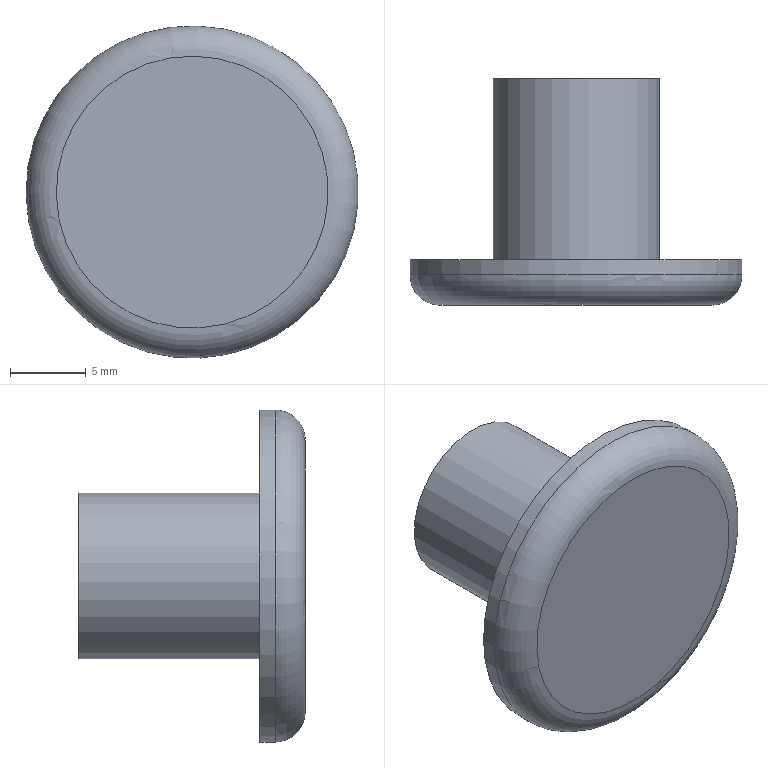Component | NX | PISTON_PIN_PLUG | 1 solid | 6 faces | box 22 x 15 x 22 mm | volume 2224 mm3 | plane 3 | cylinder 2 | torus 1 | commonest cylinder face diameters 11 x1 22 x1
STEP:
#1=CARTESIAN_POINT('',(0.,0.,0.));
#2=DIRECTION('',(0.,0.,1.));
#3=DIRECTION('',(1.,0.,0.));
#4=AXIS2_PLACEMENT_3D('',#1,#2,#3);
#5=CARTESIAN_POINT('',(63.57,-28.,-211.548));
#6=VERTEX_POINT('',#5);
#7=CARTESIAN_POINT('',(69.007,-28.,-212.381));
#8=DIRECTION('',(0.,-1.,0.));
#9=DIRECTION('',(-0.9885,0.,0.1514));
#10=AXIS2_PLACEMENT_3D('',#7,#8,#9);
#11=CIRCLE('',#10,5.5);
#12=CARTESIAN_POINT('',(69.007,-28.,-212.381));
#13=DIRECTION('',(0.,-1.,0.));
#14=DIRECTION('',(-0.9885,0.,0.1514));
#15=AXIS2_PLACEMENT_3D('',#12,#13,#14);
#16=PLANE('',#15);
#17=CARTESIAN_POINT('',(0.,0.));
#18=DIRECTION('',(1.,-0.));
#19=AXIS2_PLACEMENT_2D('',#17,#18);
#20=CIRCLE('',#19,5.5);
#21=(GEOMETRIC_REPRESENTATION_CONTEXT(2)PARAMETRIC_REPRESENTATION_CONTEXT()REPRESENTATION_CONTEXT('',''));
#22=DEFINITIONAL_REPRESENTATION('',(#20),#21);
#23=PCURVE('',#16,#22);
#24=CARTESIAN_POINT('',(69.007,-28.,-212.381));
#25=DIRECTION('',(0.,-1.,0.));
#26=DIRECTION('',(-0.9885,0.,0.1514));
#27=AXIS2_PLACEMENT_3D('',#24,#25,#26);
#28=CYLINDRICAL_SURFACE('',#27,5.5);
#29=CARTESIAN_POINT('',(0.,0.));
#30=DIRECTION('',(1.,0.));
#31=VECTOR('',#30,1.);
#32=LINE('',#29,#31);
#33=(GEOMETRIC_REPRESENTATION_CONTEXT(2)PARAMETRIC_REPRESENTATION_CONTEXT()REPRESENTATION_CONTEXT('',''));
#34=DEFINITIONAL_REPRESENTATION('',(#32),#33);
#35=PCURVE('',#28,#34);
#36=SURFACE_CURVE('',#11,(#23,#35),.PCURVE_S1.);
#37=EDGE_CURVE('',#6,#6,#36,.T.);
#38=ORIENTED_EDGE('',*,*,#37,.F.);
#39=EDGE_LOOP('',(#38));
#40=FACE_BOUND('',#39,.T.);
#41=ADVANCED_FACE('',(#40),#16,.F.);
#42=ORIENTED_EDGE('',*,*,#37,.T.);
#43=CARTESIAN_POINT('',(63.57,-40.,-211.548));
#44=VERTEX_POINT('',#43);
#45=CARTESIAN_POINT('',(63.57,-28.,-211.548));
#46=CARTESIAN_POINT('',(63.57,-40.,-211.548));
#47=B_SPLINE_CURVE_WITH_KNOTS('',1,(#45,#46),.UNSPECIFIED.,.F.,.F.,(2,2),(0.,12.),.PIECEWISE_BEZIER_KNOTS.);
#48=CARTESIAN_POINT('',(6.283,0.));
#49=DIRECTION('',(0.,1.));
#50=VECTOR('',#49,1.);
#51=LINE('',#48,#50);
#52=(GEOMETRIC_REPRESENTATION_CONTEXT(2)PARAMETRIC_REPRESENTATION_CONTEXT()REPRESENTATION_CONTEXT('',''));
#53=DEFINITIONAL_REPRESENTATION('',(#51),#52);
#54=PCURVE('',#28,#53);
#55=CARTESIAN_POINT('',(0.,0.));
#56=DIRECTION('',(0.,1.));
#57=VECTOR('',#56,1.);
#58=LINE('',#55,#57);
#59=(GEOMETRIC_REPRESENTATION_CONTEXT(2)PARAMETRIC_REPRESENTATION_CONTEXT()REPRESENTATION_CONTEXT('',''));
#60=DEFINITIONAL_REPRESENTATION('',(#58),#59);
#61=PCURVE('',#28,#60);
#62=SEAM_CURVE('',#47,(#54,#61),.PCURVE_S1.);
#63=EDGE_CURVE('',#6,#44,#62,.T.);
#64=ORIENTED_EDGE('',*,*,#63,.T.);
#65=CARTESIAN_POINT('',(69.007,-40.,-212.381));
#66=DIRECTION('',(0.,-1.,0.));
#67=DIRECTION('',(-0.9885,0.,0.1514));
#68=AXIS2_PLACEMENT_3D('',#65,#66,#67);
#69=CIRCLE('',#68,5.5);
#70=CARTESIAN_POINT('',(0.,12.));
#71=DIRECTION('',(1.,0.));
#72=VECTOR('',#71,1.);
#73=LINE('',#70,#72);
#74=(GEOMETRIC_REPRESENTATION_CONTEXT(2)PARAMETRIC_REPRESENTATION_CONTEXT()REPRESENTATION_CONTEXT('',''));
#75=DEFINITIONAL_REPRESENTATION('',(#73),#74);
#76=PCURVE('',#28,#75);
#77=CARTESIAN_POINT('',(58.133,-40.,-210.716));
#78=DIRECTION('',(0.,1.,0.));
#79=DIRECTION('',(0.9885,0.,-0.1514));
#80=AXIS2_PLACEMENT_3D('',#77,#78,#79);
#81=PLANE('',#80);
#82=CARTESIAN_POINT('',(5.5,0.));
#83=CARTESIAN_POINT('',(5.5,9.526));
#84=CARTESIAN_POINT('',(13.75,4.763));
#85=CARTESIAN_POINT('',(22.,0.));
#86=CARTESIAN_POINT('',(13.75,-4.763));
#87=CARTESIAN_POINT('',(5.5,-9.526));
#88=CARTESIAN_POINT('',(5.5,0.));
#89=(BOUNDED_CURVE()B_SPLINE_CURVE(2,(#82,#83,#84,#85,#86,#87,#88),.UNSPECIFIED.,.T.,.F.)B_SPLINE_CURVE_WITH_KNOTS((1,2,2,2,2,1),(-2.094,0.,2.094,4.189,6.283,8.378),.UNSPECIFIED.)CURVE()GEOMETRIC_REPRESENTATION_ITEM()RATIONAL_B_SPLINE_CURVE((1.,0.5,1.,0.5,1.,0.5,1.))REPRESENTATION_ITEM(''));
#90=(GEOMETRIC_REPRESENTATION_CONTEXT(2)PARAMETRIC_REPRESENTATION_CONTEXT()REPRESENTATION_CONTEXT('',''));
#91=DEFINITIONAL_REPRESENTATION('',(#89),#90);
#92=PCURVE('',#81,#91);
#93=SURFACE_CURVE('',#69,(#76,#92),.PCURVE_S1.);
#94=EDGE_CURVE('',#44,#44,#93,.T.);
#95=ORIENTED_EDGE('',*,*,#94,.F.);
#96=ORIENTED_EDGE('',*,*,#63,.F.);
#97=EDGE_LOOP('',(#42,#64,#95,#96));
#98=FACE_BOUND('',#97,.T.);
#99=ADVANCED_FACE('',(#98),#28,.T.);
#100=ORIENTED_EDGE('',*,*,#94,.T.);
#101=EDGE_LOOP('',(#100));
#102=FACE_BOUND('',#101,.T.);
#103=CARTESIAN_POINT('',(58.133,-40.,-210.716));
#104=VERTEX_POINT('',#103);
#105=CARTESIAN_POINT('',(69.007,-40.,-212.381));
#106=DIRECTION('',(0.,-1.,0.));
#107=DIRECTION('',(-0.9885,0.,0.1514));
#108=AXIS2_PLACEMENT_3D('',#105,#106,#107);
#109=CIRCLE('',#108,11.);
#110=CARTESIAN_POINT('',(0.,0.));
#111=CARTESIAN_POINT('',(0.,19.053));
#112=CARTESIAN_POINT('',(16.5,9.526));
#113=CARTESIAN_POINT('',(33.,0.));
#114=CARTESIAN_POINT('',(16.5,-9.526));
#115=CARTESIAN_POINT('',(0.,-19.053));
#116=CARTESIAN_POINT('',(0.,0.));
#117=(BOUNDED_CURVE()B_SPLINE_CURVE(2,(#110,#111,#112,#113,#114,#115,#116),.UNSPECIFIED.,.T.,.F.)B_SPLINE_CURVE_WITH_KNOTS((1,2,2,2,2,1),(-2.094,0.,2.094,4.189,6.283,8.378),.UNSPECIFIED.)CURVE()GEOMETRIC_REPRESENTATION_ITEM()RATIONAL_B_SPLINE_CURVE((1.,0.5,1.,0.5,1.,0.5,1.))REPRESENTATION_ITEM(''));
#118=(GEOMETRIC_REPRESENTATION_CONTEXT(2)PARAMETRIC_REPRESENTATION_CONTEXT()REPRESENTATION_CONTEXT('',''));
#119=DEFINITIONAL_REPRESENTATION('',(#117),#118);
#120=PCURVE('',#81,#119);
#121=CARTESIAN_POINT('',(69.007,-28.,-212.381));
#122=DIRECTION('',(0.,-1.,0.));
#123=DIRECTION('',(-0.9885,0.,0.1514));
#124=AXIS2_PLACEMENT_3D('',#121,#122,#123);
#125=CYLINDRICAL_SURFACE('',#124,11.);
#126=CARTESIAN_POINT('',(0.,12.));
#127=DIRECTION('',(1.,0.));
#128=VECTOR('',#127,1.);
#129=LINE('',#126,#128);
#130=(GEOMETRIC_REPRESENTATION_CONTEXT(2)PARAMETRIC_REPRESENTATION_CONTEXT()REPRESENTATION_CONTEXT('',''));
#131=DEFINITIONAL_REPRESENTATION('',(#129),#130);
#132=PCURVE('',#125,#131);
#133=SURFACE_CURVE('',#109,(#120,#132),.PCURVE_S1.);
#134=EDGE_CURVE('',#104,#104,#133,.T.);
#135=ORIENTED_EDGE('',*,*,#134,.F.);
#136=EDGE_LOOP('',(#135));
#137=FACE_BOUND('',#136,.T.);
#138=ADVANCED_FACE('',(#102,#137),#81,.T.);
#139=ORIENTED_EDGE('',*,*,#134,.T.);
#140=CARTESIAN_POINT('',(58.133,-41.,-210.716));
#141=VERTEX_POINT('',#140);
#142=CARTESIAN_POINT('',(58.133,-40.,-210.716));
#143=CARTESIAN_POINT('',(58.133,-41.,-210.716));
#144=B_SPLINE_CURVE_WITH_KNOTS('',1,(#142,#143),.UNSPECIFIED.,.F.,.F.,(2,2),(12.,13.),.PIECEWISE_BEZIER_KNOTS.);
#145=CARTESIAN_POINT('',(6.283,0.));
#146=DIRECTION('',(0.,1.));
#147=VECTOR('',#146,1.);
#148=LINE('',#145,#147);
#149=(GEOMETRIC_REPRESENTATION_CONTEXT(2)PARAMETRIC_REPRESENTATION_CONTEXT()REPRESENTATION_CONTEXT('',''));
#150=DEFINITIONAL_REPRESENTATION('',(#148),#149);
#151=PCURVE('',#125,#150);
#152=CARTESIAN_POINT('',(0.,0.));
#153=DIRECTION('',(0.,1.));
#154=VECTOR('',#153,1.);
#155=LINE('',#152,#154);
#156=(GEOMETRIC_REPRESENTATION_CONTEXT(2)PARAMETRIC_REPRESENTATION_CONTEXT()REPRESENTATION_CONTEXT('',''));
#157=DEFINITIONAL_REPRESENTATION('',(#155),#156);
#158=PCURVE('',#125,#157);
#159=SEAM_CURVE('',#144,(#151,#158),.PCURVE_S1.);
#160=EDGE_CURVE('',#104,#141,#159,.T.);
#161=ORIENTED_EDGE('',*,*,#160,.T.);
#162=CARTESIAN_POINT('',(69.007,-41.,-212.381));
#163=DIRECTION('',(0.,-1.,0.));
#164=DIRECTION('',(-0.9885,0.,0.1514));
#165=AXIS2_PLACEMENT_3D('',#162,#163,#164);
#166=CIRCLE('',#165,11.);
#167=CARTESIAN_POINT('',(0.,13.));
#168=DIRECTION('',(1.,0.));
#169=VECTOR('',#168,1.);
#170=LINE('',#167,#169);
#171=(GEOMETRIC_REPRESENTATION_CONTEXT(2)PARAMETRIC_REPRESENTATION_CONTEXT()REPRESENTATION_CONTEXT('',''));
#172=DEFINITIONAL_REPRESENTATION('',(#170),#171);
#173=PCURVE('',#125,#172);
#174=CARTESIAN_POINT('',(69.007,-41.,-212.381));
#175=DIRECTION('',(0.,-1.,0.));
#176=DIRECTION('',(-0.9885,0.,0.1514));
#177=AXIS2_PLACEMENT_3D('',#174,#175,#176);
#178=TOROIDAL_SURFACE('',#177,9.,2.);
#179=CARTESIAN_POINT('',(0.,6.283));
#180=DIRECTION('',(1.,0.));
#181=VECTOR('',#180,1.);
#182=LINE('',#179,#181);
#183=(GEOMETRIC_REPRESENTATION_CONTEXT(2)PARAMETRIC_REPRESENTATION_CONTEXT()REPRESENTATION_CONTEXT('',''));
#184=DEFINITIONAL_REPRESENTATION('',(#182),#183);
#185=PCURVE('',#178,#184);
#186=SURFACE_CURVE('',#166,(#173,#185),.PCURVE_S1.);
#187=EDGE_CURVE('',#141,#141,#186,.T.);
#188=ORIENTED_EDGE('',*,*,#187,.F.);
#189=ORIENTED_EDGE('',*,*,#160,.F.);
#190=EDGE_LOOP('',(#139,#161,#188,#189));
#191=FACE_BOUND('',#190,.T.);
#192=ADVANCED_FACE('',(#191),#125,.T.);
#193=ORIENTED_EDGE('',*,*,#187,.T.);
#194=CARTESIAN_POINT('',(60.11,-43.,-211.019));
#195=VERTEX_POINT('',#194);
#196=CARTESIAN_POINT('',(58.133,-41.,-210.716));
#197=CARTESIAN_POINT('',(58.133,-41.535,-210.716));
#198=CARTESIAN_POINT('',(58.301,-42.055,-210.742));
#199=CARTESIAN_POINT('',(58.624,-42.504,-210.791));
#200=CARTESIAN_POINT('',(59.067,-42.83,-210.859));
#201=CARTESIAN_POINT('',(59.582,-43.,-210.938));
#202=CARTESIAN_POINT('',(60.11,-43.,-211.019));
#203=(BOUNDED_CURVE()B_SPLINE_CURVE(6,(#196,#197,#198,#199,#200,#201,#202),.UNSPECIFIED.,.F.,.F.)B_SPLINE_CURVE_WITH_KNOTS((7,7),(0.,1.571),.PIECEWISE_BEZIER_KNOTS.)CURVE()GEOMETRIC_REPRESENTATION_ITEM()RATIONAL_B_SPLINE_CURVE((1.031,1.01,0.9979,0.994,0.9979,1.01,1.031))REPRESENTATION_ITEM(''));
#204=CARTESIAN_POINT('',(6.283,6.283));
#205=DIRECTION('',(0.,1.));
#206=VECTOR('',#205,1.);
#207=LINE('',#204,#206);
#208=(GEOMETRIC_REPRESENTATION_CONTEXT(2)PARAMETRIC_REPRESENTATION_CONTEXT()REPRESENTATION_CONTEXT('',''));
#209=DEFINITIONAL_REPRESENTATION('',(#207),#208);
#210=PCURVE('',#178,#209);
#211=CARTESIAN_POINT('',(0.,6.283));
#212=DIRECTION('',(0.,1.));
#213=VECTOR('',#212,1.);
#214=LINE('',#211,#213);
#215=(GEOMETRIC_REPRESENTATION_CONTEXT(2)PARAMETRIC_REPRESENTATION_CONTEXT()REPRESENTATION_CONTEXT('',''));
#216=DEFINITIONAL_REPRESENTATION('',(#214),#215);
#217=PCURVE('',#178,#216);
#218=SEAM_CURVE('',#203,(#210,#217),.PCURVE_S1.);
#219=EDGE_CURVE('',#141,#195,#218,.T.);
#220=ORIENTED_EDGE('',*,*,#219,.T.);
#221=CARTESIAN_POINT('',(69.007,-43.,-212.381));
#222=DIRECTION('',(0.,-1.,0.));
#223=DIRECTION('',(-0.9885,0.,0.1514));
#224=AXIS2_PLACEMENT_3D('',#221,#222,#223);
#225=CIRCLE('',#224,9.);
#226=CARTESIAN_POINT('',(0.,7.854));
#227=DIRECTION('',(1.,0.));
#228=VECTOR('',#227,1.);
#229=LINE('',#226,#228);
#230=(GEOMETRIC_REPRESENTATION_CONTEXT(2)PARAMETRIC_REPRESENTATION_CONTEXT()REPRESENTATION_CONTEXT('',''));
#231=DEFINITIONAL_REPRESENTATION('',(#229),#230);
#232=PCURVE('',#178,#231);
#233=CARTESIAN_POINT('',(69.007,-43.,-212.381));
#234=DIRECTION('',(0.,-1.,0.));
#235=DIRECTION('',(-0.9885,0.,0.1514));
#236=AXIS2_PLACEMENT_3D('',#233,#234,#235);
#237=PLANE('',#236);
#238=CARTESIAN_POINT('',(0.,0.));
#239=DIRECTION('',(1.,0.));
#240=AXIS2_PLACEMENT_2D('',#238,#239);
#241=CIRCLE('',#240,9.);
#242=(GEOMETRIC_REPRESENTATION_CONTEXT(2)PARAMETRIC_REPRESENTATION_CONTEXT()REPRESENTATION_CONTEXT('',''));
#243=DEFINITIONAL_REPRESENTATION('',(#241),#242);
#244=PCURVE('',#237,#243);
#245=SURFACE_CURVE('',#225,(#232,#244),.PCURVE_S1.);
#246=EDGE_CURVE('',#195,#195,#245,.T.);
#247=ORIENTED_EDGE('',*,*,#246,.F.);
#248=ORIENTED_EDGE('',*,*,#219,.F.);
#249=EDGE_LOOP('',(#193,#220,#247,#248));
#250=FACE_BOUND('',#249,.T.);
#251=ADVANCED_FACE('',(#250),#178,.T.);
#252=ORIENTED_EDGE('',*,*,#246,.T.);
#253=EDGE_LOOP('',(#252));
#254=FACE_BOUND('',#253,.T.);
#255=ADVANCED_FACE('',(#254),#237,.T.);
#256=CLOSED_SHELL('',(#41,#99,#138,#192,#251,#255));
#257=MANIFOLD_SOLID_BREP('',#256);
#258=(LENGTH_UNIT()NAMED_UNIT(*)SI_UNIT(.MILLI.,.METRE.));
#259=UNCERTAINTY_MEASURE_WITH_UNIT(LENGTH_MEASURE(0.00001),#258,'','');
#260=(NAMED_UNIT(*)PLANE_ANGLE_UNIT()SI_UNIT($,.RADIAN.));
#261=(NAMED_UNIT(*)SI_UNIT($,.STERADIAN.)SOLID_ANGLE_UNIT());
#262=(GEOMETRIC_REPRESENTATION_CONTEXT(3)GLOBAL_UNCERTAINTY_ASSIGNED_CONTEXT((#259))GLOBAL_UNIT_ASSIGNED_CONTEXT((#258,#260,#261))REPRESENTATION_CONTEXT('',''));
#263=ADVANCED_BREP_SHAPE_REPRESENTATION('',(#4,#257),#262);